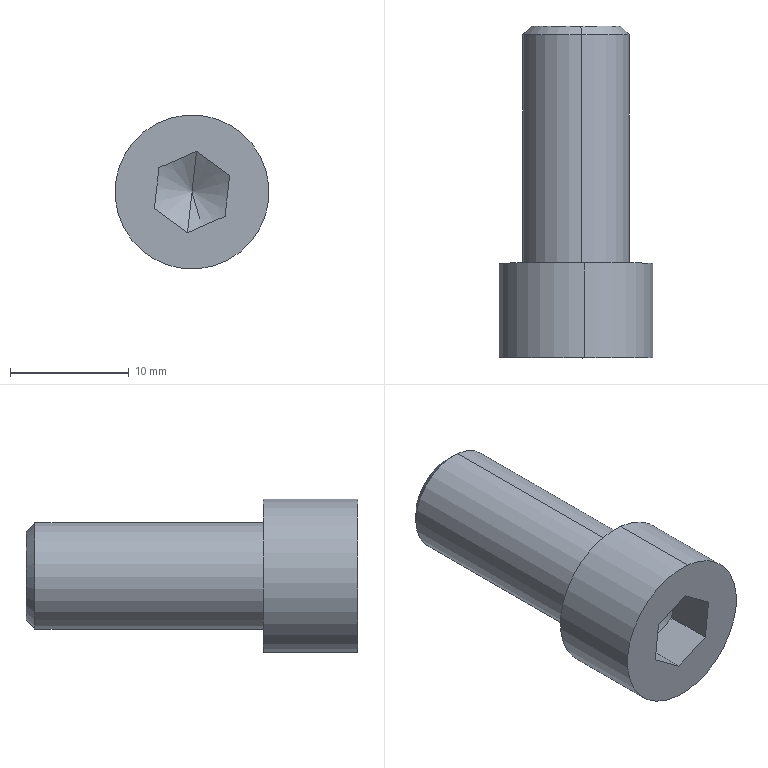Component | SolidWorks | 11-1 | 1 solid | 31 faces | volume 2139 mm3 | plane 21 | cylinder 6 | cone 4 | commonest cylinder face diameters 6.928 x2 9 x2 13 x2